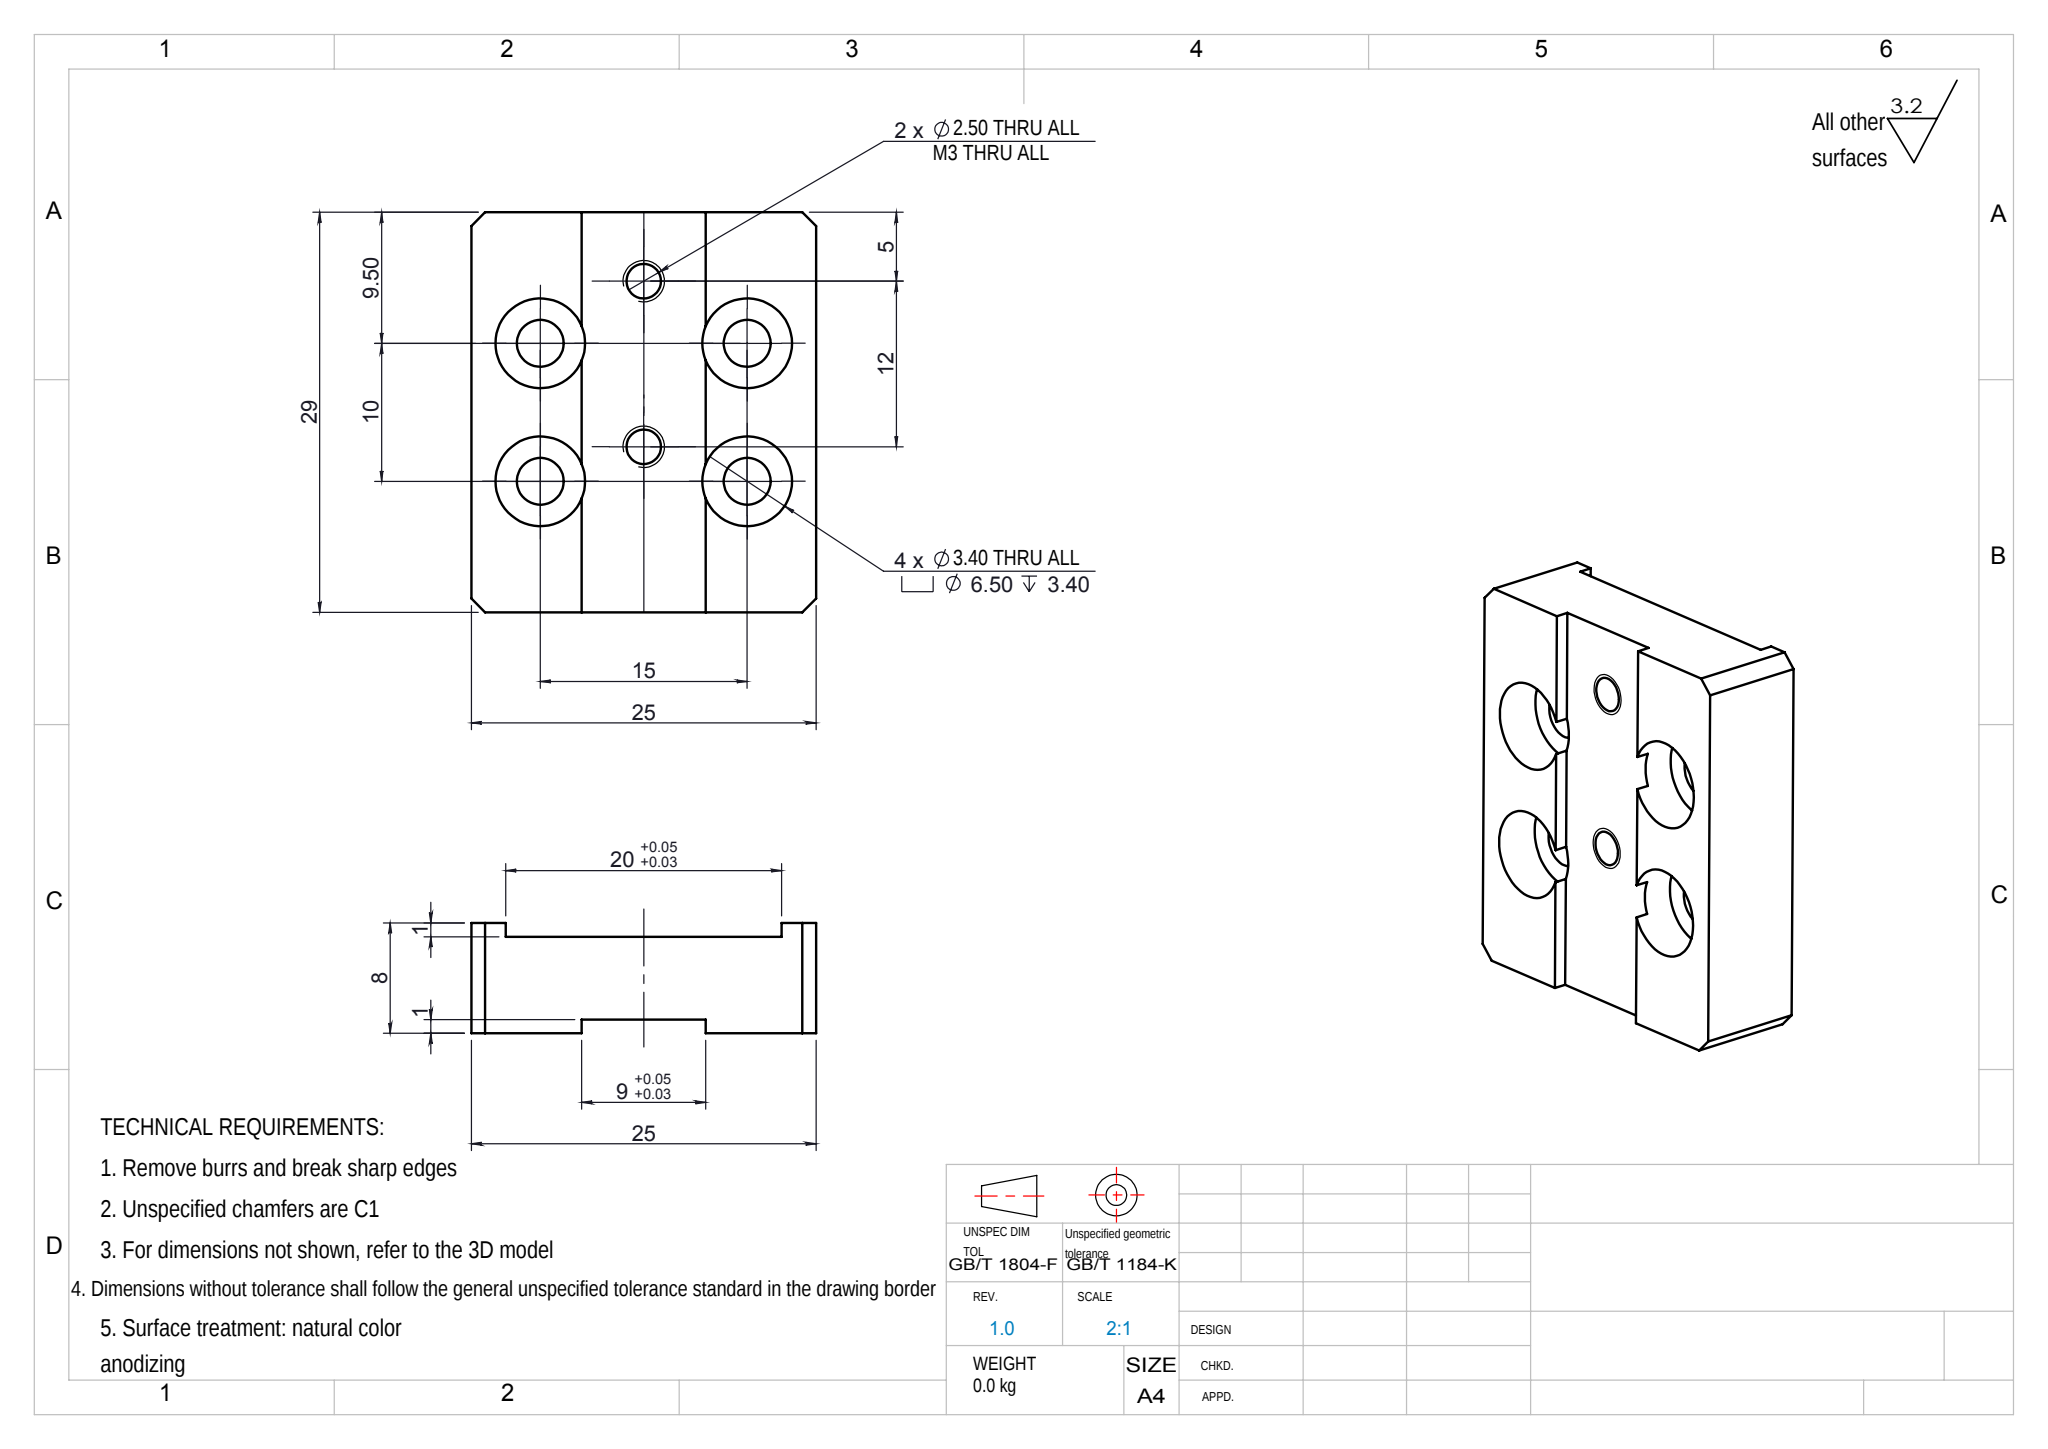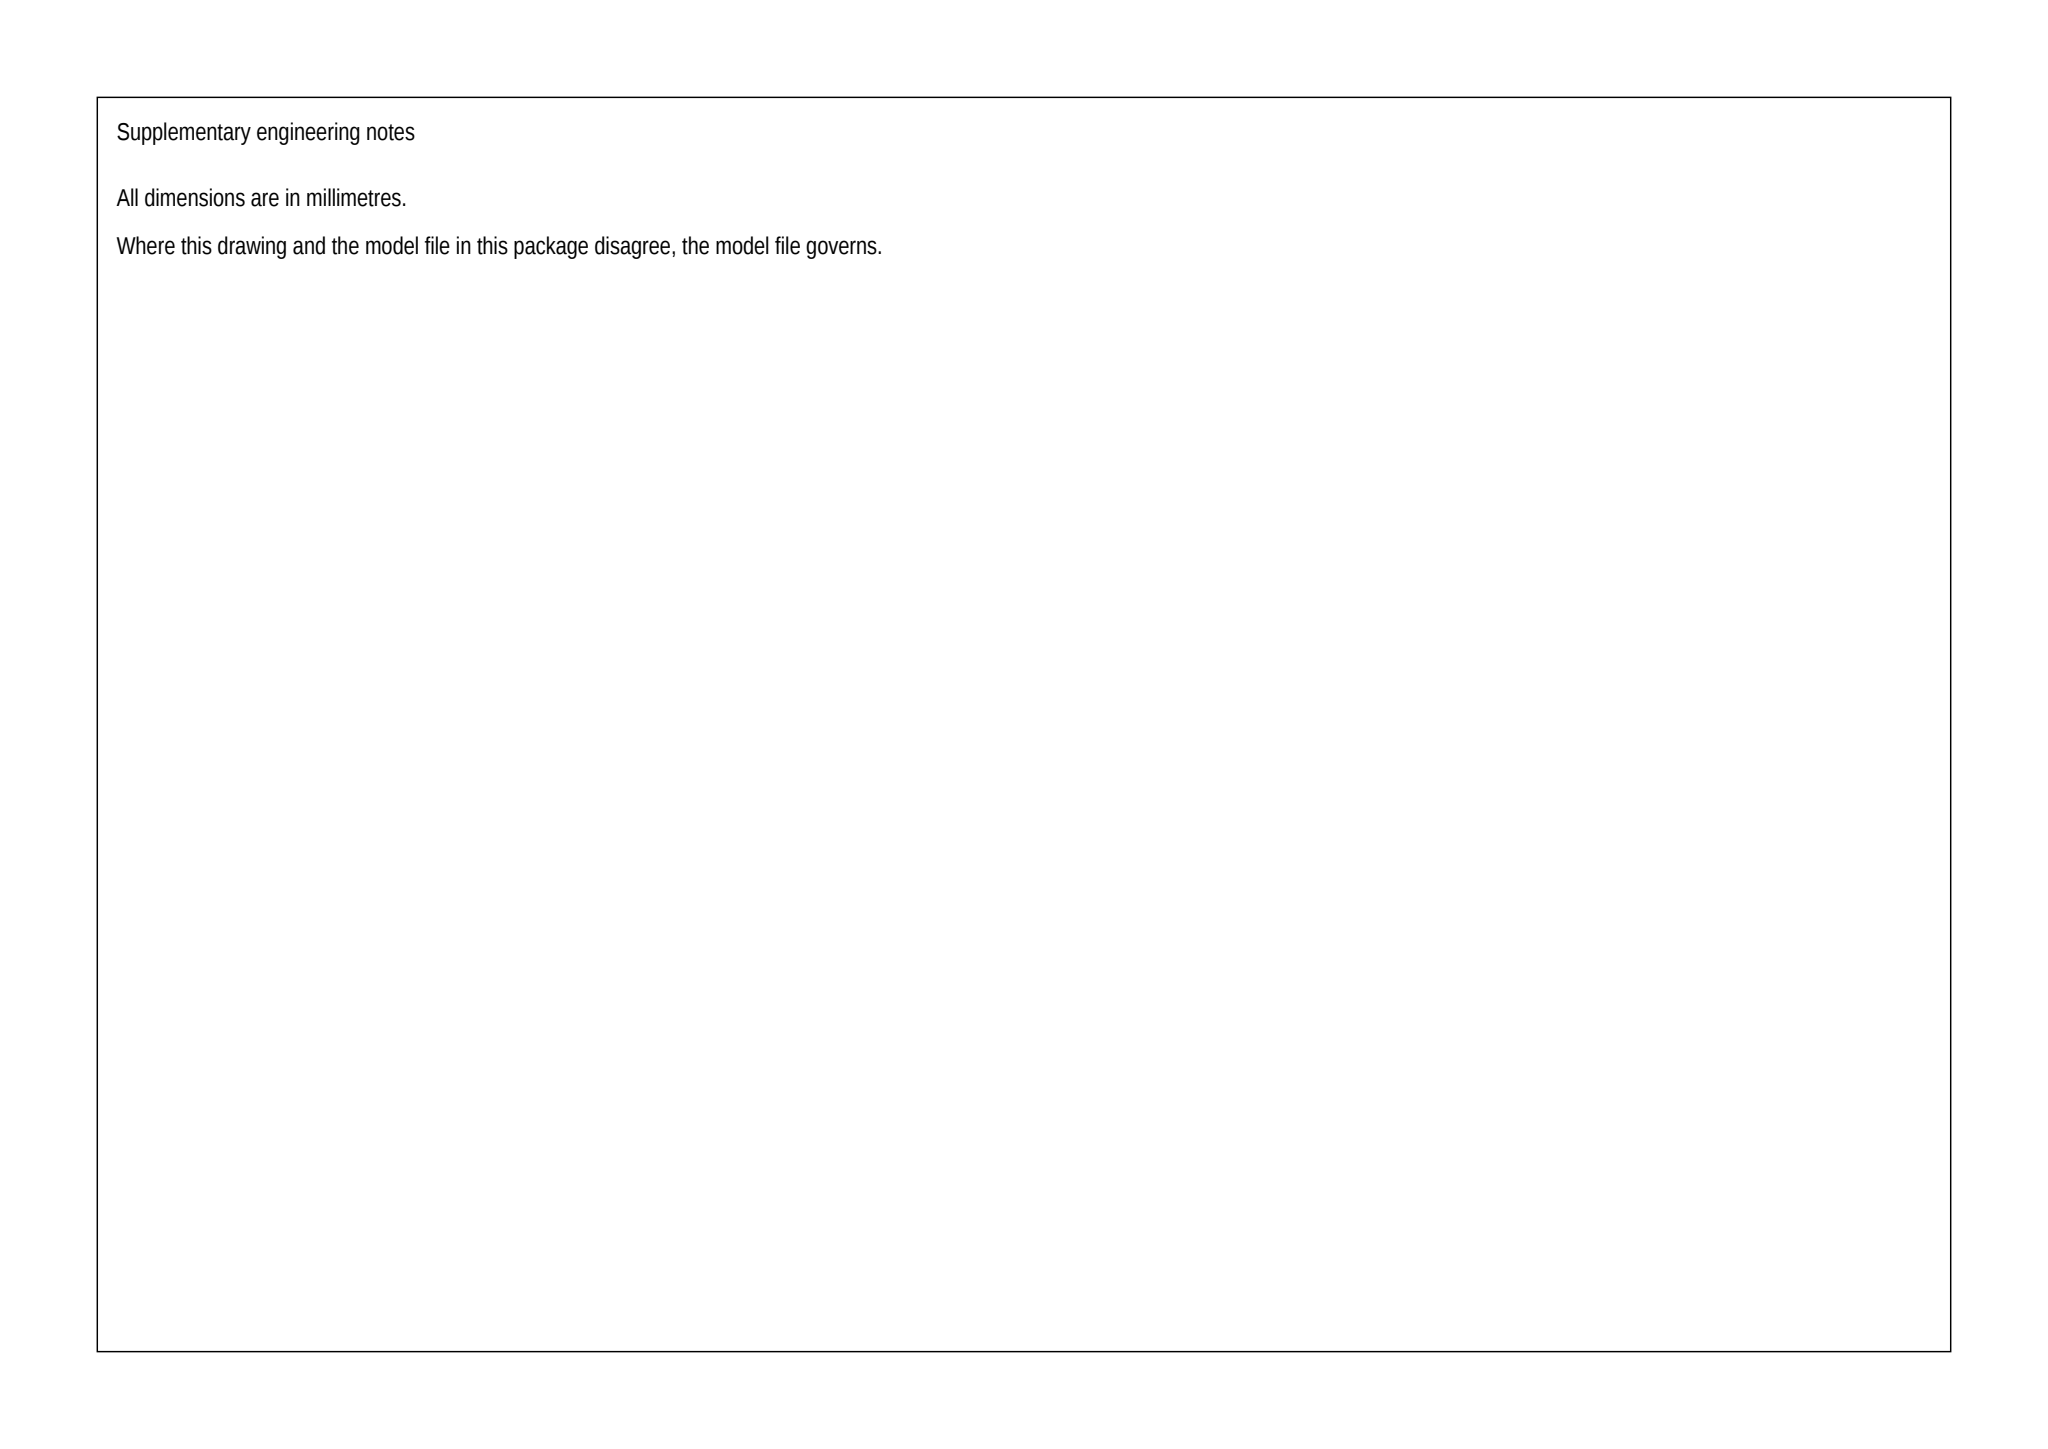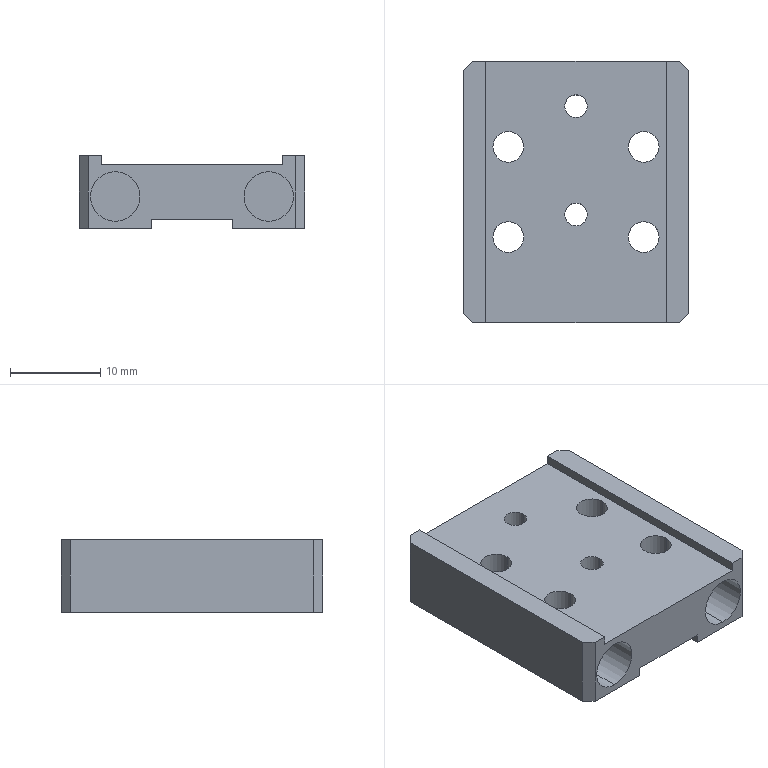Part | SolidWorks | mm | 1 solid | 52 faces | box 25 x 29 x 8 mm | volume 4066 mm3 | plane 28 | cylinder 24 | commonest cylinder face diameters 6.5 x8 3.4 x8 2.5 x4 5.5 x4
Drawing notes:
TOP STEPS 1 DP x 2.5 WIDE EA END, LEAVES 20 RAISED FACE | from the solid: x-planes 2.5 and 22.5 (20 span) on 25 width; z 7.0 vs top 8.0 = 1 DP
BTM RECESS 9 WIDE x 1 DP, CTRD ON 25 WIDTH, 8 FROM EA EDGE | from the solid: x-planes 8.0/17.0 (9 wide, ctrd at 12.5); z-planes 0.0 and 1.0
4 x CBORE HOLES ON CL 5 FROM EA SIDE EDGE OF 25 WIDTH | from the solid: Ø3.4/Ø6.5 cyls at x=5.0 and x=20.0 (25-20=5)
2 x M3 THRU ON CTR BAND CL, 12.5 FROM SIDE EDGE | from the solid: Ø2.5 cyls at x=12.5 (ctr of 25 width), y=12.0 and 24.0
2 x Ø5.5 DP 5 IN 25 x 8 BOTTOM EDGE FACE (Y=0), AXIS PERP FACE | from the solid: cylinders dia 5.5, axis y, length 5.0, starting at y=0 face (y-plane 0, bbox 25x29x8)
Ø5.5 EDGE HOLES: AXES 3.5 UP FROM BOTTOM FACE | from the solid: cylinders dia 5.5 pos z=3.5 from z=0 face (8 thk)
Ø5.5 EDGE HOLES AT 4 AND 21 FROM LH EDGE (17 APART) | from the solid: cylinders dia 5.5 at x=4.0 and x=21.0 from x=0 face of 25 width
build123d program:
from build123d import *

# Parameters (mm, degrees)
SKETCH1_W                                       = 25
SKETCH1_H                                       = 29
BOSS_EXTRUDE1_DEPTH                             = 8
SKETCH2_W                                       = 20
SKETCH2_H                                       = 29
CUT_EXTRUDE1_DEPTH                              = 1
M3_HEX_SOCKET_HEAD_CAP_SCREW_CBORE1_D           = 3.4
M3_HEX_SOCKET_HEAD_CAP_SCREW_CBORE1_CBORE_D     = 6.5
M3_HEX_SOCKET_HEAD_CAP_SCREW_CBORE1_CBORE_DEPTH = 3.4
SKETCH5_W                                       = 9
SKETCH5_H                                       = 29
CUT_EXTRUDE2_DEPTH                              = 1
SKETCH8_R                                       = 2.75
CUT_EXTRUDE3_DEPTH                              = 5
M3_TAPPED_HOLE1_D                               = 2.5
CHAMFER1_SIZE                                   = 1


with BuildPart() as part:
    # Sketch1 → Boss-Extrude1 (new body)
    with BuildSketch(Plane.XY):
        Rectangle(SKETCH1_W, SKETCH1_H)
    extrude(amount=BOSS_EXTRUDE1_DEPTH)

    # Sketch2 → Cut-Extrude1 (cut)
    with BuildSketch(Plane.XY.offset(8)):
        Rectangle(SKETCH2_W, SKETCH2_H)
    extrude(amount=-CUT_EXTRUDE1_DEPTH, mode=Mode.SUBTRACT)

    # M3 Hex Socket Head Cap Screw CBORE1 (through all)
    with Locations(Plane(origin=(0, 0, 0), x_dir=(-1, 0, 0), z_dir=(0, 0, -1))):
        with Locations((-7.5, 5), (-7.5, -5), (7.5, -5), (7.5, 5)):
            CounterBoreHole(M3_HEX_SOCKET_HEAD_CAP_SCREW_CBORE1_D / 2, M3_HEX_SOCKET_HEAD_CAP_SCREW_CBORE1_CBORE_D / 2, M3_HEX_SOCKET_HEAD_CAP_SCREW_CBORE1_CBORE_DEPTH)

    # Sketch5 → Cut-Extrude2 (cut)
    with BuildSketch(Plane(origin=(0, 0, 0), x_dir=(-1, 0, 0), z_dir=(0, 0, -1))):
        Rectangle(SKETCH5_W, SKETCH5_H)
    extrude(amount=-CUT_EXTRUDE2_DEPTH, mode=Mode.SUBTRACT)

    # Sketch8 → Cut-Extrude3 (cut)
    with BuildSketch(Plane.XZ.offset(14.5)):
        with Locations(Location((-8.5, 3.5, 0), (0, 0, 270))):
            Circle(SKETCH8_R)
        with Locations(Location((8.5, 3.5, 0), (0, 0, 90))):
            Circle(SKETCH8_R)
    extrude(amount=-CUT_EXTRUDE3_DEPTH, mode=Mode.SUBTRACT)

    # M3 Tapped Hole1 (through all)
    with Locations(Plane(origin=(0, 0, 1), x_dir=(-1, 0, 0), z_dir=(0, 0, -1))):
        with Locations((0, -2.5), (0, 9.5)):
            Hole(M3_TAPPED_HOLE1_D / 2)

    # Chamfer1
    chamfer1_edges = [part.edges().sort_by_distance(p)[0] for p in [
        (12.5, -14.5, 4),
        (-12.5, -14.5, 4),
        (-12.5, 14.5, 4),
        (12.5, 14.5, 4),
    ]]
    chamfer(chamfer1_edges, length=CHAMFER1_SIZE)


solid = part.part